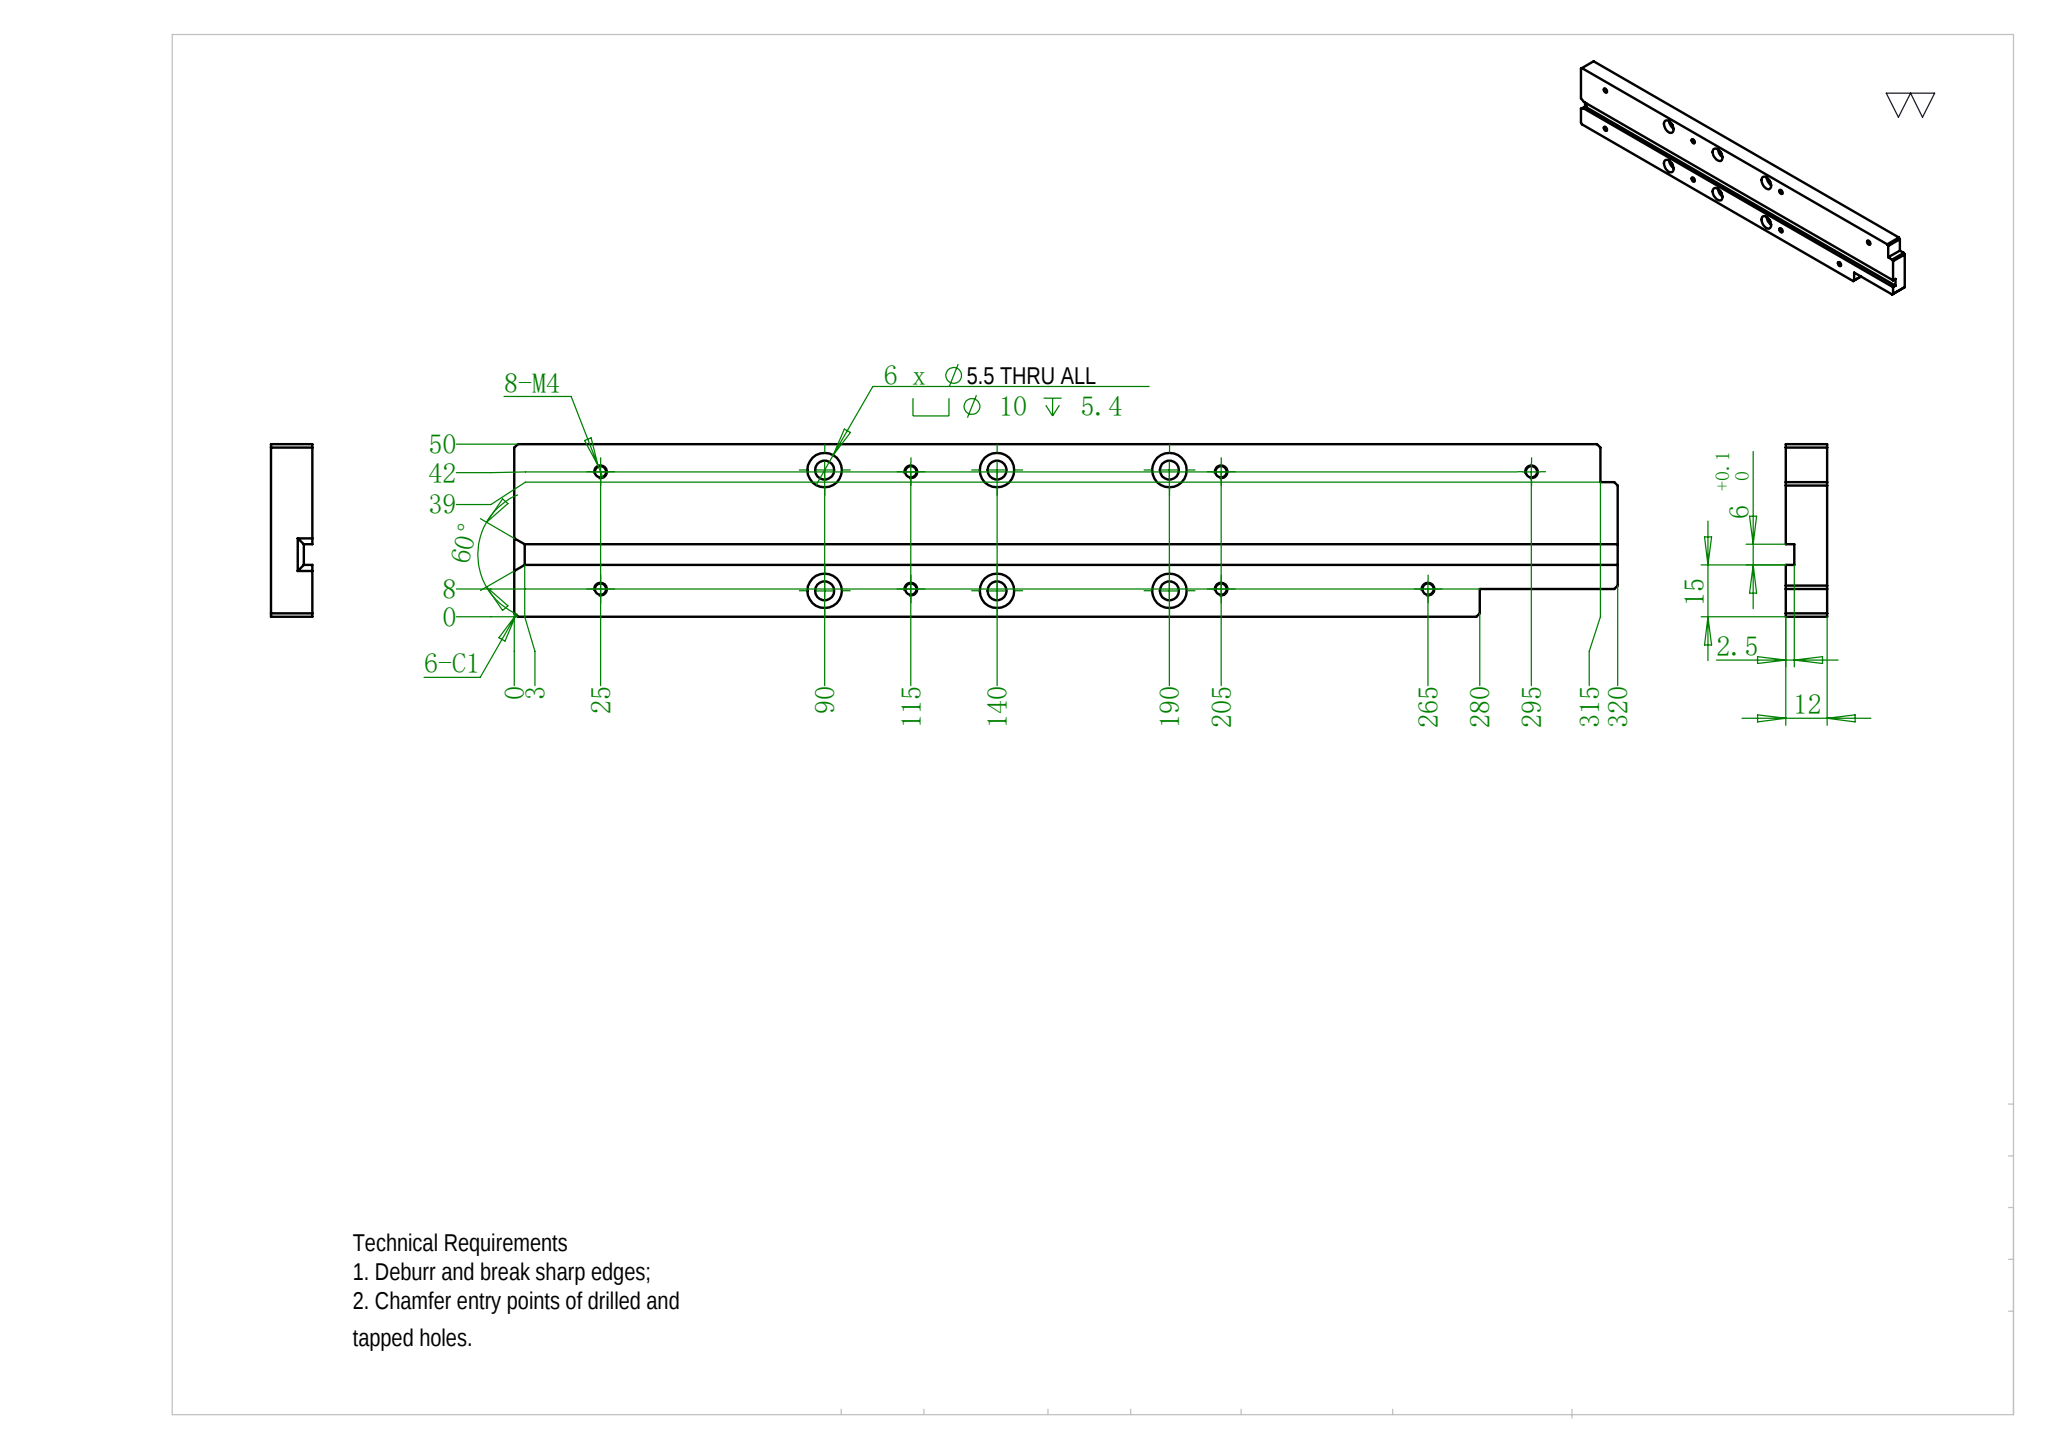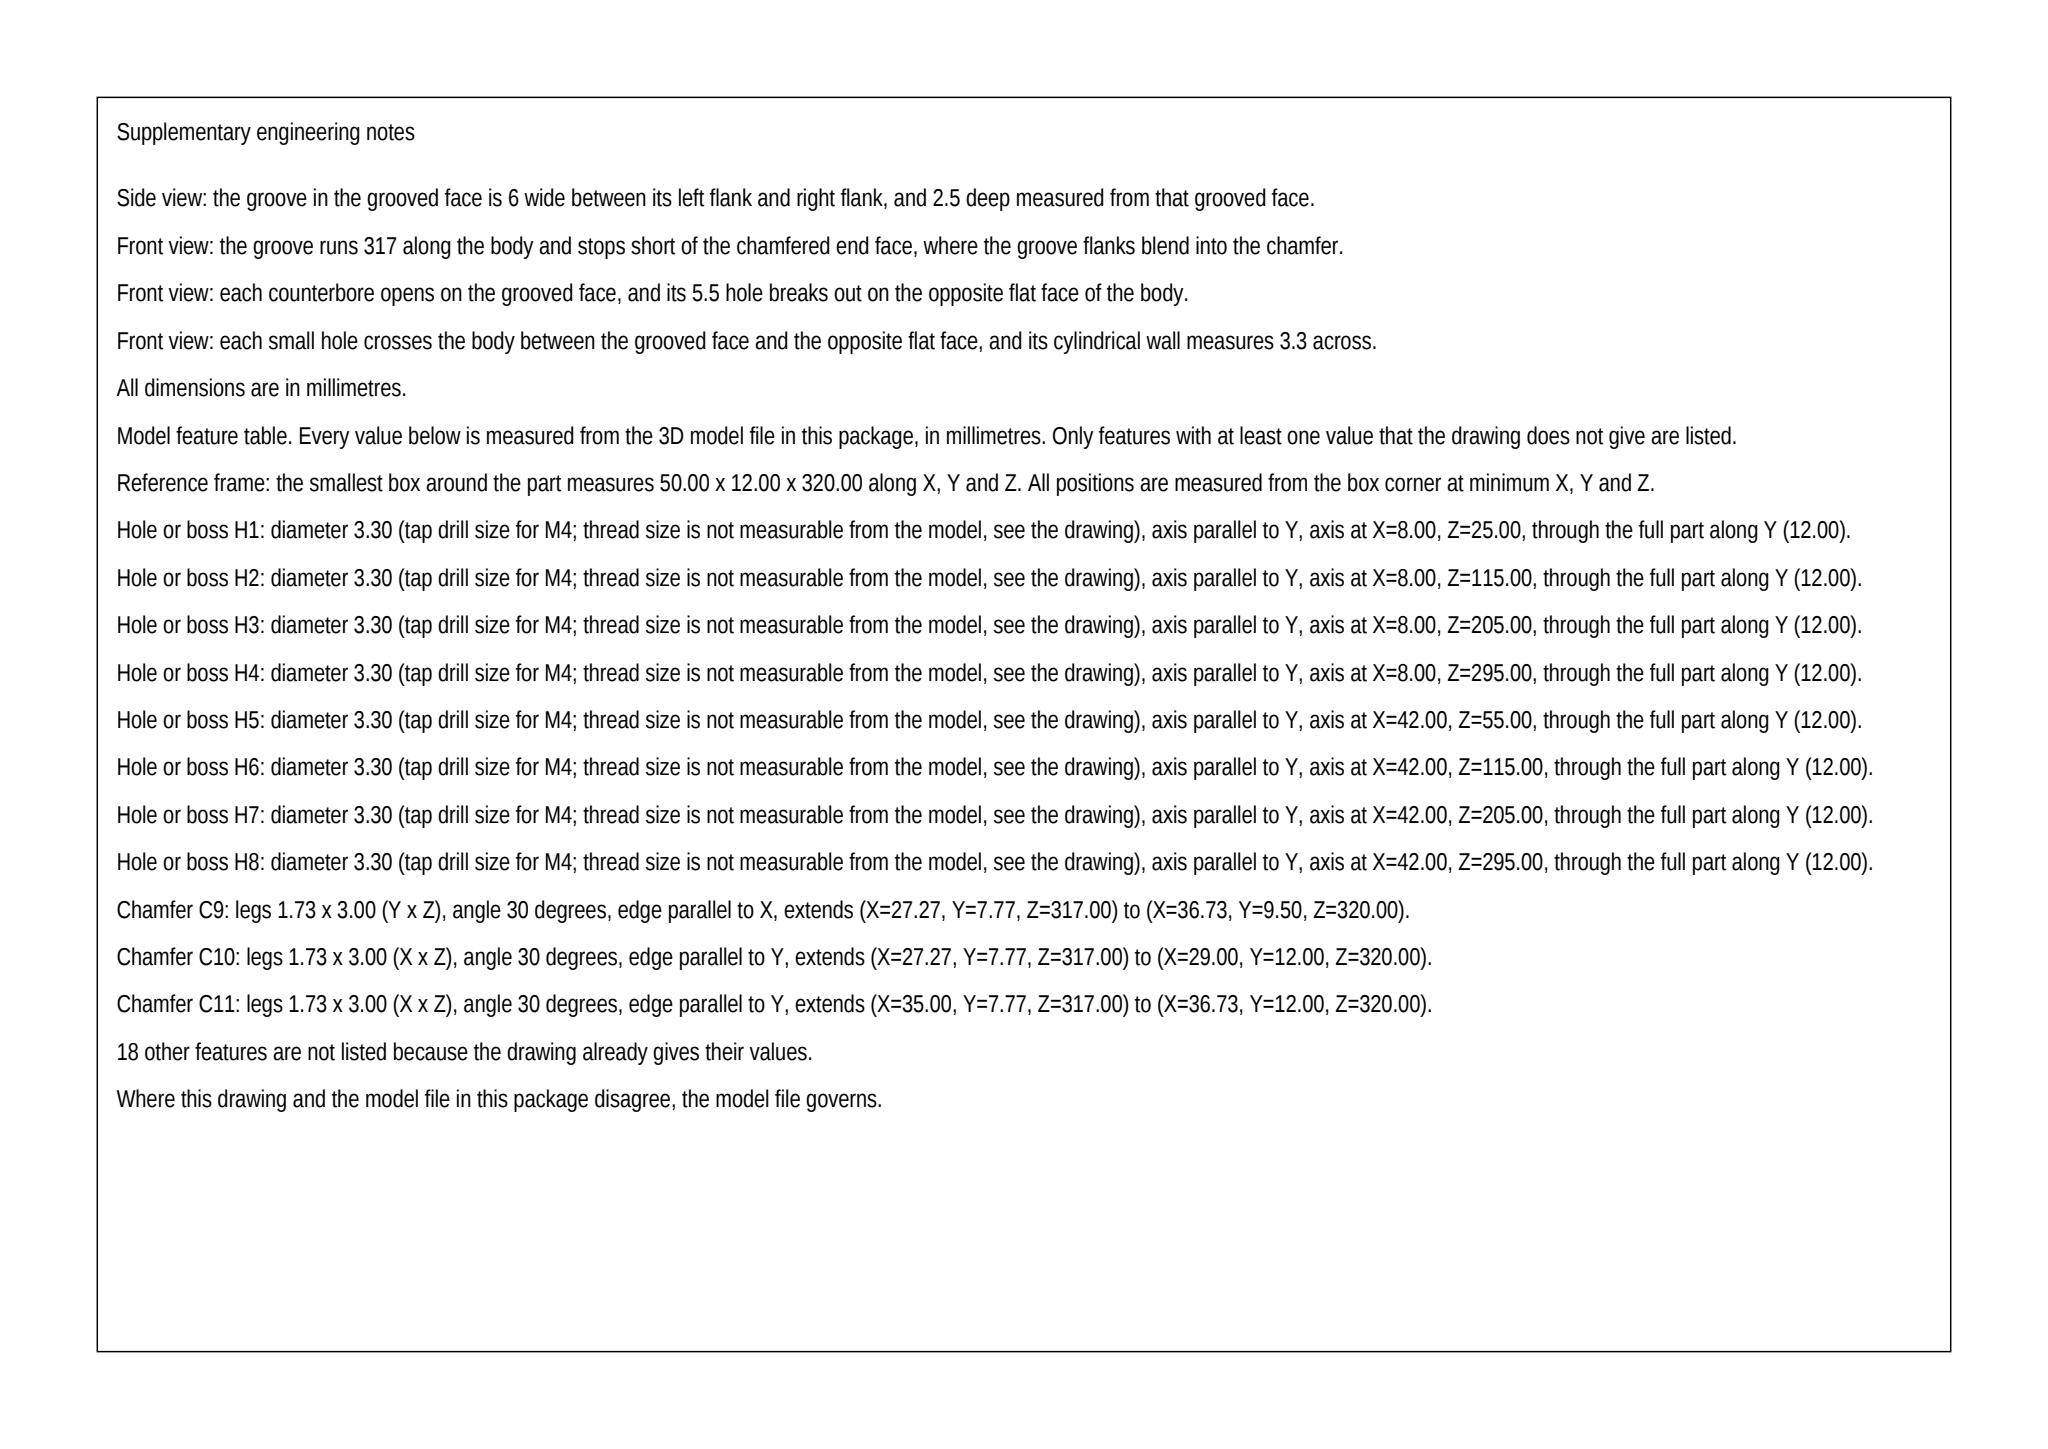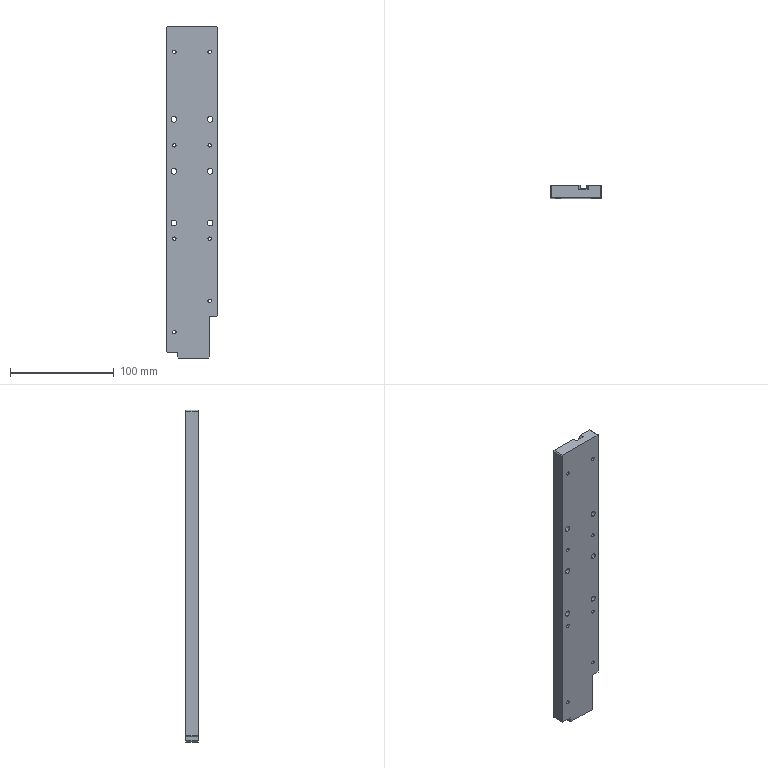Part | SolidWorks | mm | 1 solid | 69 faces | box 50 x 12 x 320 mm | volume 178323 mm3 | cylinder 40 | plane 29 | commonest cylinder face diameters 3.3 x16 10 x12 5.5 x12
build123d program:
from build123d import *
from OCP.BRepFilletAPI import BRepFilletAPI_MakeChamfer

# Parameters (mm, degrees)
SKETCH1_W                                       = 50
SKETCH1_H                                       = 12
BOSS_EXTRUDE1_DEPTH                             = 320
SKETCH17_W                                      = 6
SKETCH17_H                                      = 2.5
CUT_EXTRUDE1_DEPTH                              = 325.105
M5_HEX_SOCKET_HEAD_CAP_SCREW_CBORE1_D           = 5.5
M5_HEX_SOCKET_HEAD_CAP_SCREW_CBORE1_CBORE_D     = 10
M5_HEX_SOCKET_HEAD_CAP_SCREW_CBORE1_CBORE_DEPTH = 5.4
M4_TAPPED_HOLE3_D                               = 3.3
SKETCH24_W                                      = 11
SKETCH24_H                                      = 5
CUT_EXTRUDE4_DEPTH                              = 325.105
CHAMFER1_SIZE                                   = 3
CHAMFER1_SIZE2                                  = 1.732
CHAMFER2_SIZE                                   = 1
SKETCH26_W                                      = 8
SKETCH26_H                                      = 40
CUT_EXTRUDE6_DEPTH                              = 325.105
CHAMFER3_SIZE                                   = 1


with BuildPart() as part:
    # Sketch1 → Boss-Extrude1 (new body)
    with BuildSketch(Plane.XY):
        with Locations((25, 6)):
            Rectangle(SKETCH1_W, SKETCH1_H)
    extrude(amount=BOSS_EXTRUDE1_DEPTH)

    # Sketch17 → Cut-Extrude1 (cut, through all)
    with BuildSketch(Plane.XY.offset(320)):
        with Locations((32, 10.75)):
            Rectangle(SKETCH17_W, SKETCH17_H)
    extrude(amount=-CUT_EXTRUDE1_DEPTH, mode=Mode.SUBTRACT)

    # M5 Hex Socket Head Cap Screw CBORE1 (through all)
    with Locations(Plane(origin=(0, 12, 0), x_dir=(1, 0, 0), z_dir=(0, 1, 0))):
        with Locations((7.5, -130), (7.5, -180), (7.5, -230), (42.5, -230), (42.5, -180), (42.5, -130)):
            CounterBoreHole(M5_HEX_SOCKET_HEAD_CAP_SCREW_CBORE1_D / 2, M5_HEX_SOCKET_HEAD_CAP_SCREW_CBORE1_CBORE_D / 2, M5_HEX_SOCKET_HEAD_CAP_SCREW_CBORE1_CBORE_DEPTH)

    # M4 Tapped Hole3 (through all)
    with Locations(Plane(origin=(0, 12, 0), x_dir=(1, 0, 0), z_dir=(0, 1, 0))):
        with Locations((42, -55), (8, -25), (8, -115), (42, -115), (42, -205), (8, -205), (42, -295), (8, -295)):
            Hole(M4_TAPPED_HOLE3_D / 2)

    # Sketch24 → Cut-Extrude4 (cut, through all)
    with BuildSketch(Plane(origin=(0, 12, 0), x_dir=(1, 0, 0), z_dir=(0, 1, 0))):
        with Locations((5.5, -2.5)):
            Rectangle(SKETCH24_W, SKETCH24_H)
    extrude(amount=-CUT_EXTRUDE4_DEPTH, mode=Mode.SUBTRACT)

    # Chamfer1: one chamfer whose edges measure the first distance from different faces: ONE call of the kernel's chamfer builder (chamfer() names one face for all edges)
    chamfer1_edges_1 = [part.edges().sort_by_distance(p)[0] for p in [
        (29, 10.75, 320),
    ]]
    chamfer1_side_1 = [part.faces().sort_by_distance(p)[0] for p in [
        (29, 10.75, 160),
    ]]
    chamfer1_edges_2 = [part.edges().sort_by_distance(p)[0] for p in [
        (32, 9.5, 320),
    ]]
    chamfer1_side_2 = [part.faces().sort_by_distance(p)[0] for p in [
        (32, 9.5, 160),
    ]]
    chamfer1_edges_3 = [part.edges().sort_by_distance(p)[0] for p in [
        (35, 10.75, 320),
    ]]
    chamfer1_side_3 = [part.faces().sort_by_distance(p)[0] for p in [
        (35, 10.75, 160),
    ]]
    chamfer1 = BRepFilletAPI_MakeChamfer(part.part.solid().wrapped)
    for e in chamfer1_edges_1:
        chamfer1.Add(CHAMFER1_SIZE, CHAMFER1_SIZE2, e.wrapped, chamfer1_side_1[0].wrapped)  # the first distance lies on this face
    for e in chamfer1_edges_2:
        chamfer1.Add(CHAMFER1_SIZE, CHAMFER1_SIZE2, e.wrapped, chamfer1_side_2[0].wrapped)  # the first distance lies on this face
    for e in chamfer1_edges_3:
        chamfer1.Add(CHAMFER1_SIZE, CHAMFER1_SIZE2, e.wrapped, chamfer1_side_3[0].wrapped)  # the first distance lies on this face
    add(Compound.cast(chamfer1.Shape()), mode=Mode.REPLACE)

    # Chamfer2
    chamfer2_edges = [part.edges().sort_by_distance(p)[0] for p in [
        (0, 6, 5),
        (0, 6, 320),
        (11, 6, 0),
        (50, 6, 0),
        (50, 6, 320),
    ]]
    chamfer(chamfer2_edges, length=CHAMFER2_SIZE)

    # Sketch26 → Cut-Extrude6 (cut, through all)
    with BuildSketch(Plane(origin=(0, 12, 0), x_dir=(1, 0, 0), z_dir=(0, 1, 0))):
        with Locations((46, -20)):
            Rectangle(SKETCH26_W, SKETCH26_H)
    extrude(amount=-CUT_EXTRUDE6_DEPTH, mode=Mode.SUBTRACT)

    # Chamfer3
    chamfer3_edges = [part.edges().sort_by_distance(p)[0] for p in [
        (42, 6, 0),
        (50, 6, 40),
    ]]
    chamfer(chamfer3_edges, length=CHAMFER3_SIZE)


solid = part.part